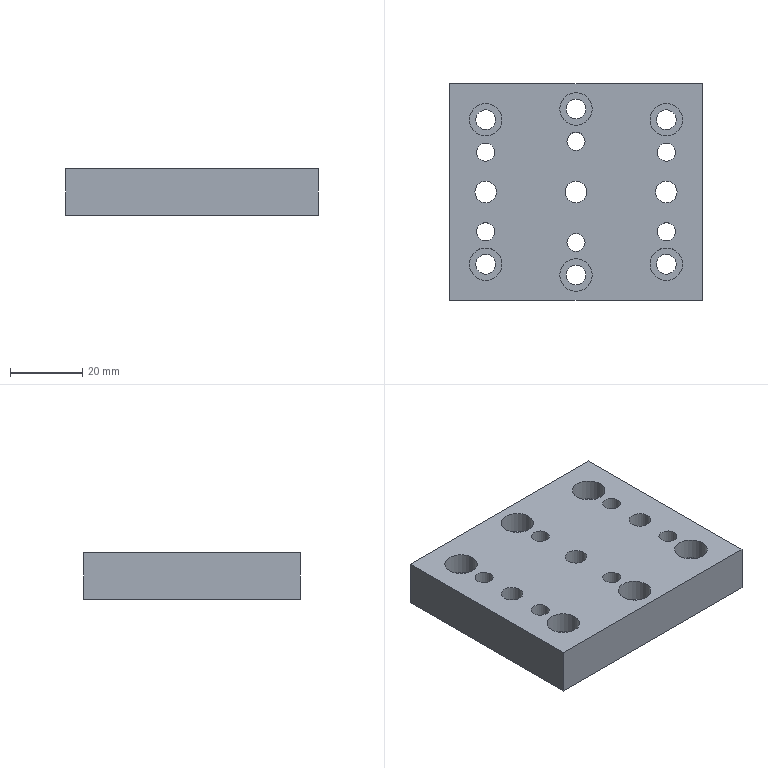Component | NX | BASE | 1 solid | 33 faces | volume 48678 mm3 | cylinder 21 | plane 12 | commonest cylinder face diameters 5.5 x6 5 x6 9 x6 6 x3